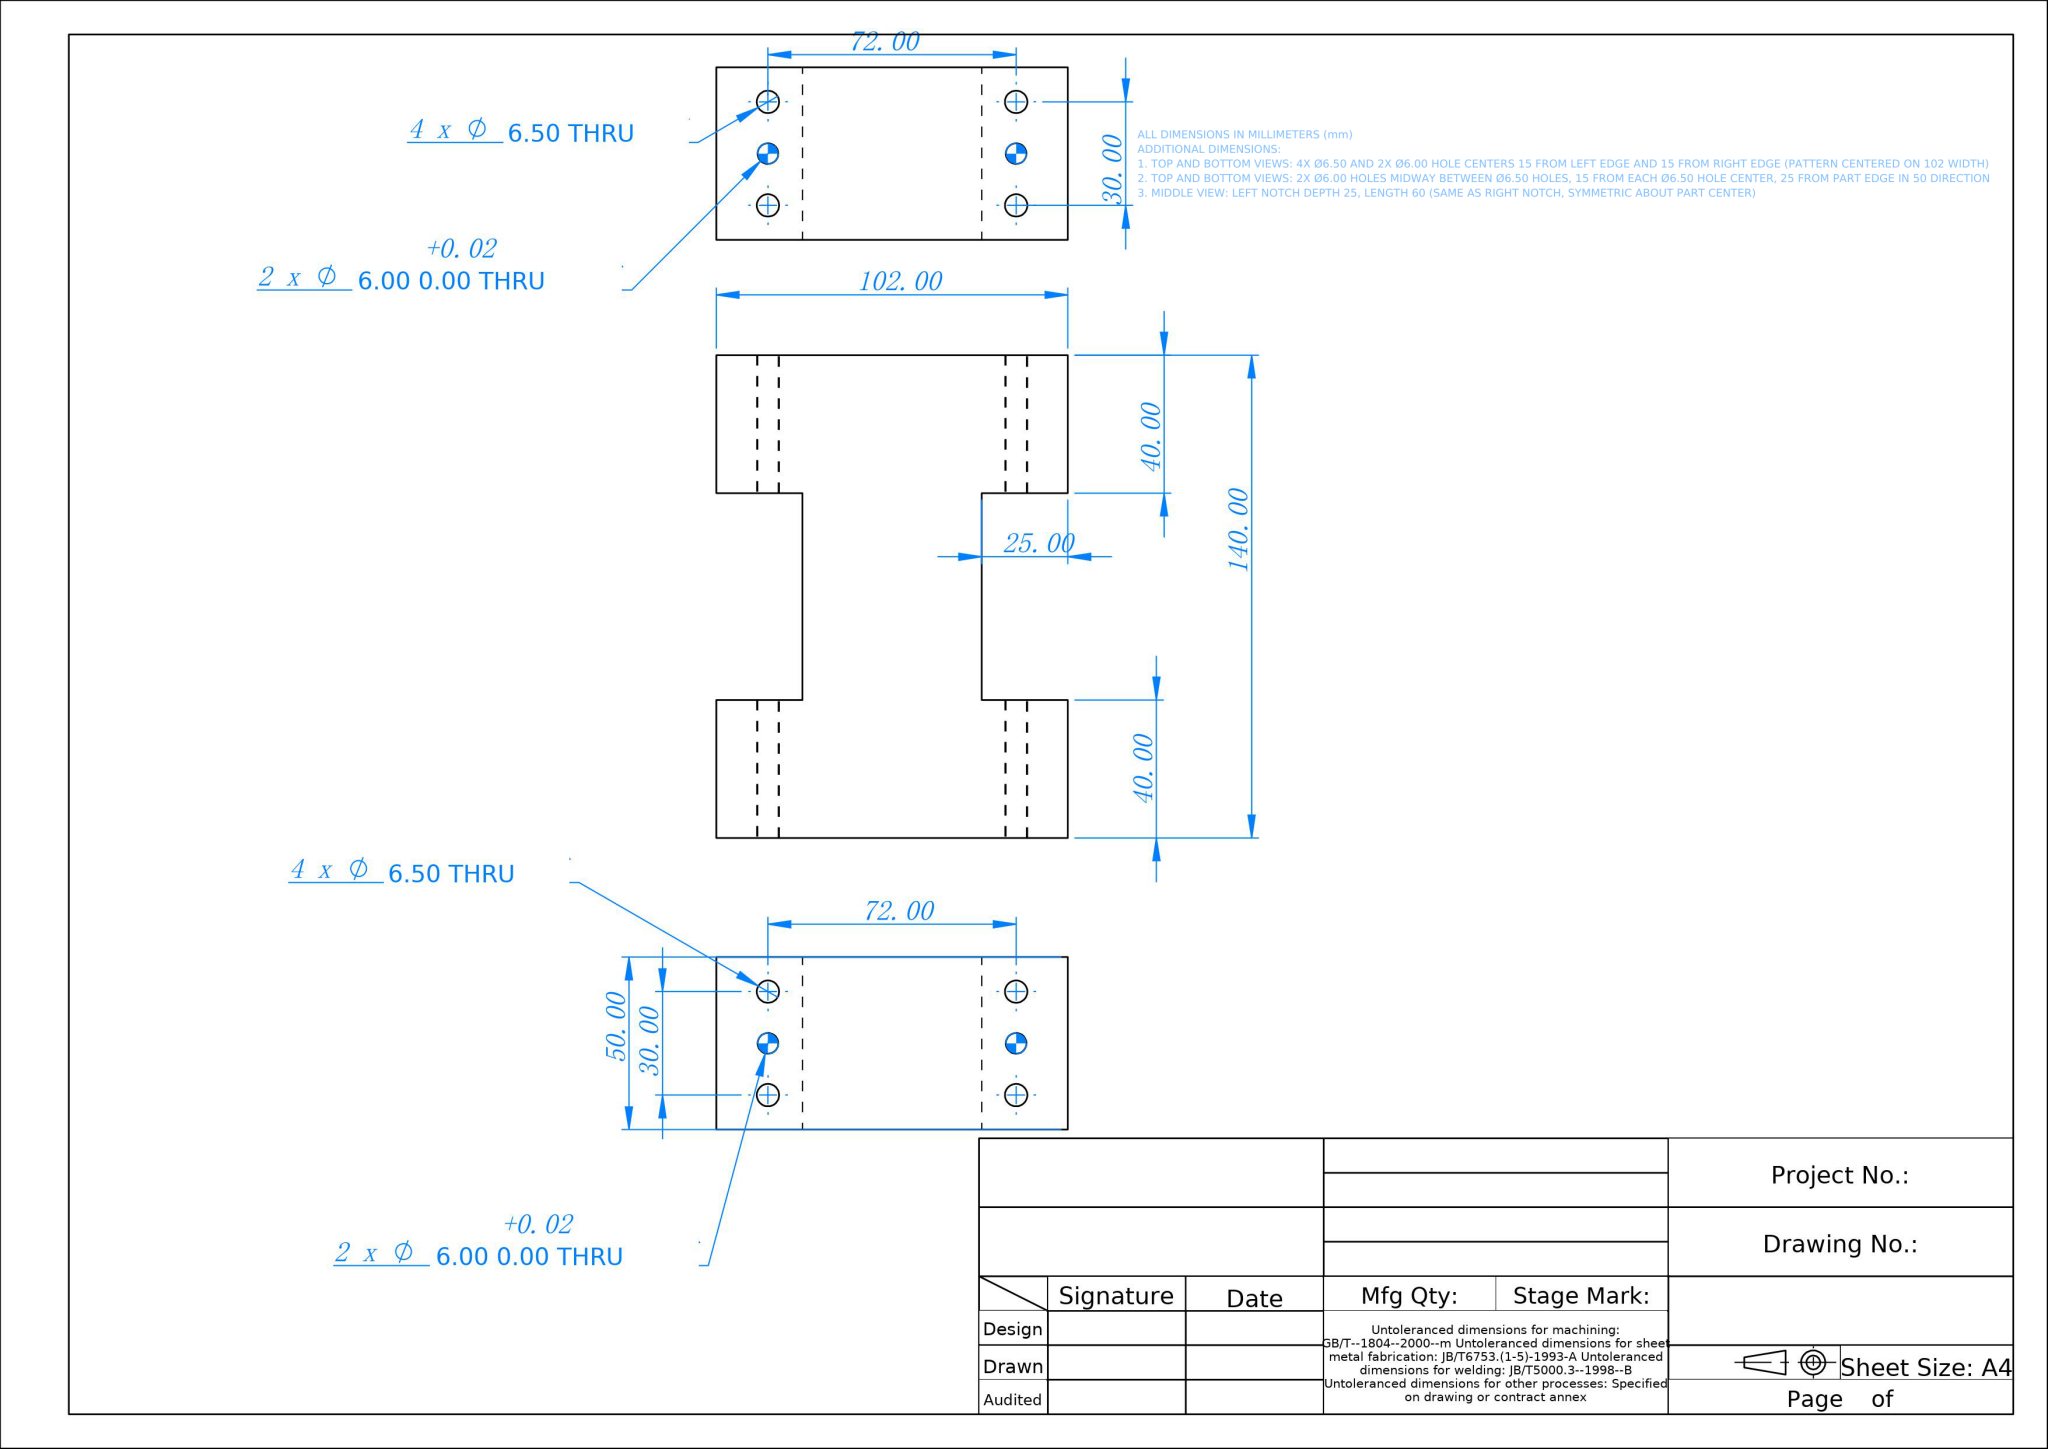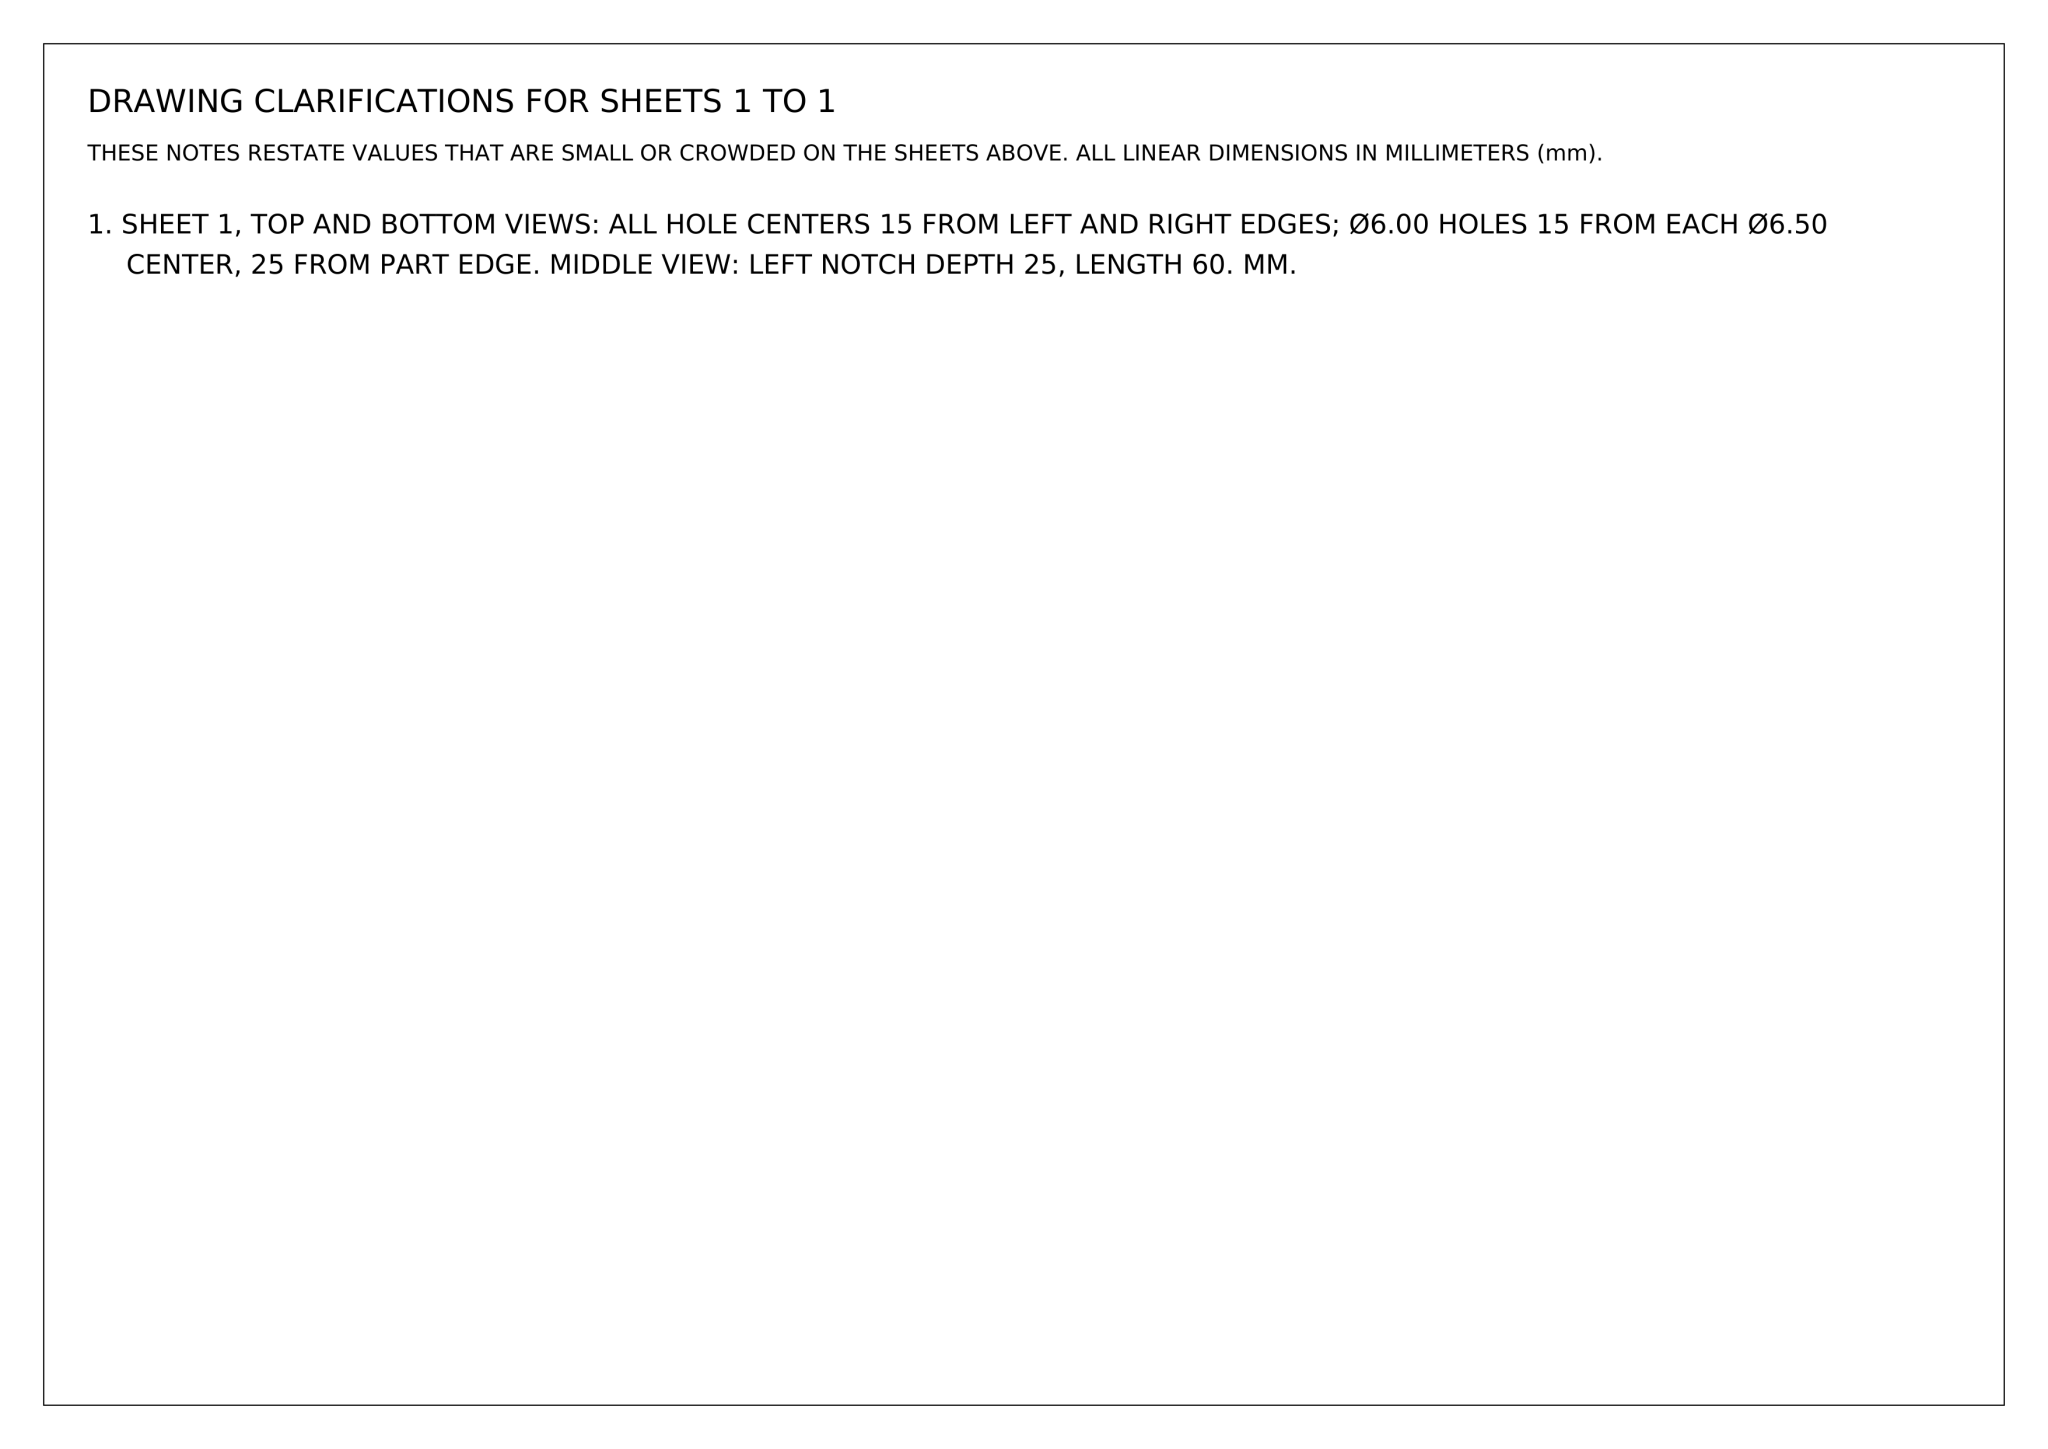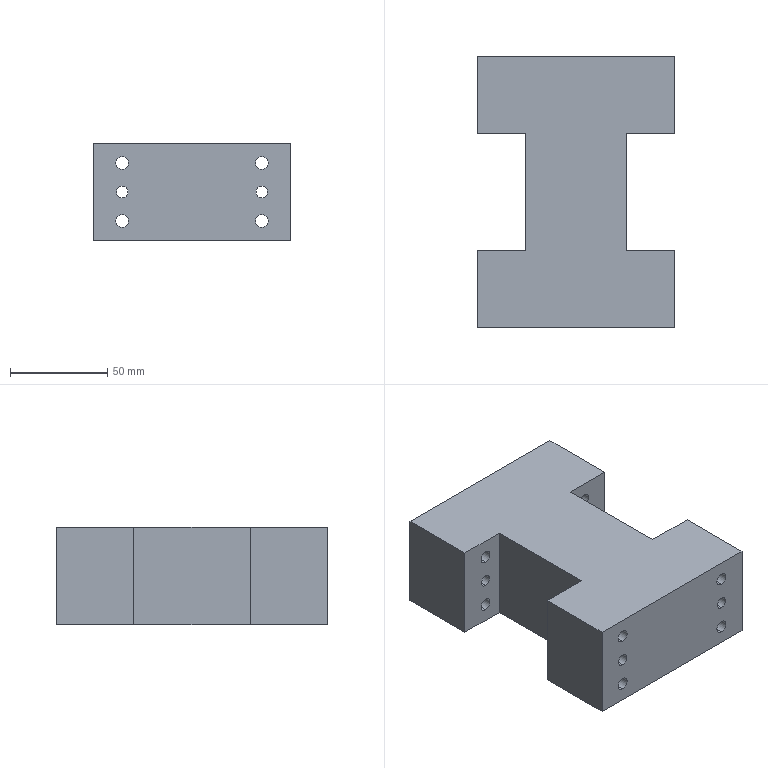Part | NX | mm | 1 solid | 38 faces | box 102 x 140 x 50 mm | volume 548858 mm3 | cylinder 24 | plane 14 | commonest cylinder face diameters 6.5 x16 6 x8